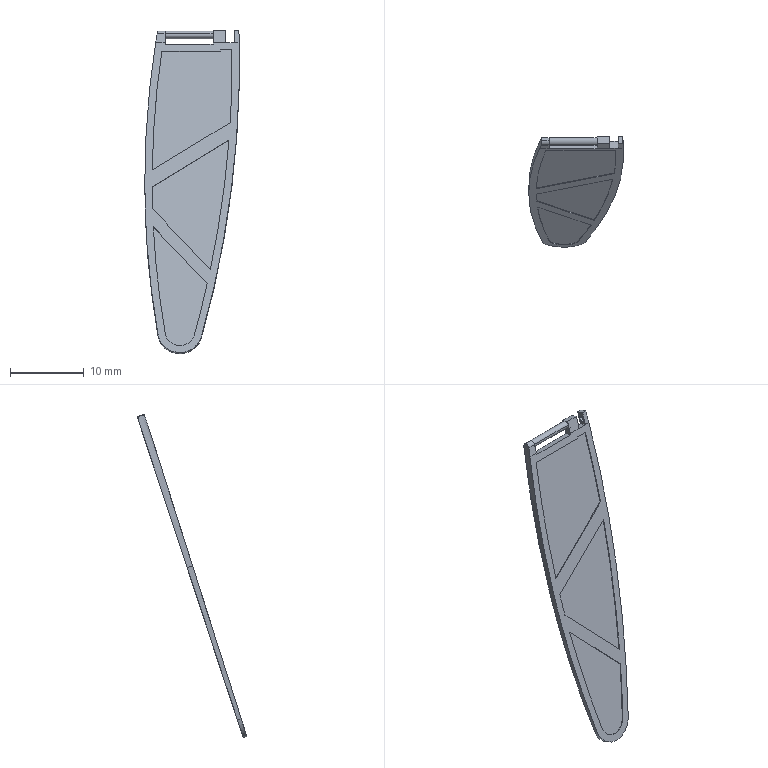Component | SolidWorks | FrontWing-4 | 1 solid | 63 faces | volume 301 mm3 | plane 37 | cylinder 24 | spline 2 | commonest cylinder face diameters 264.615 x6 298.038 x6 0.8 x4 1 x4 266.581 x2 6 x1 300 x1